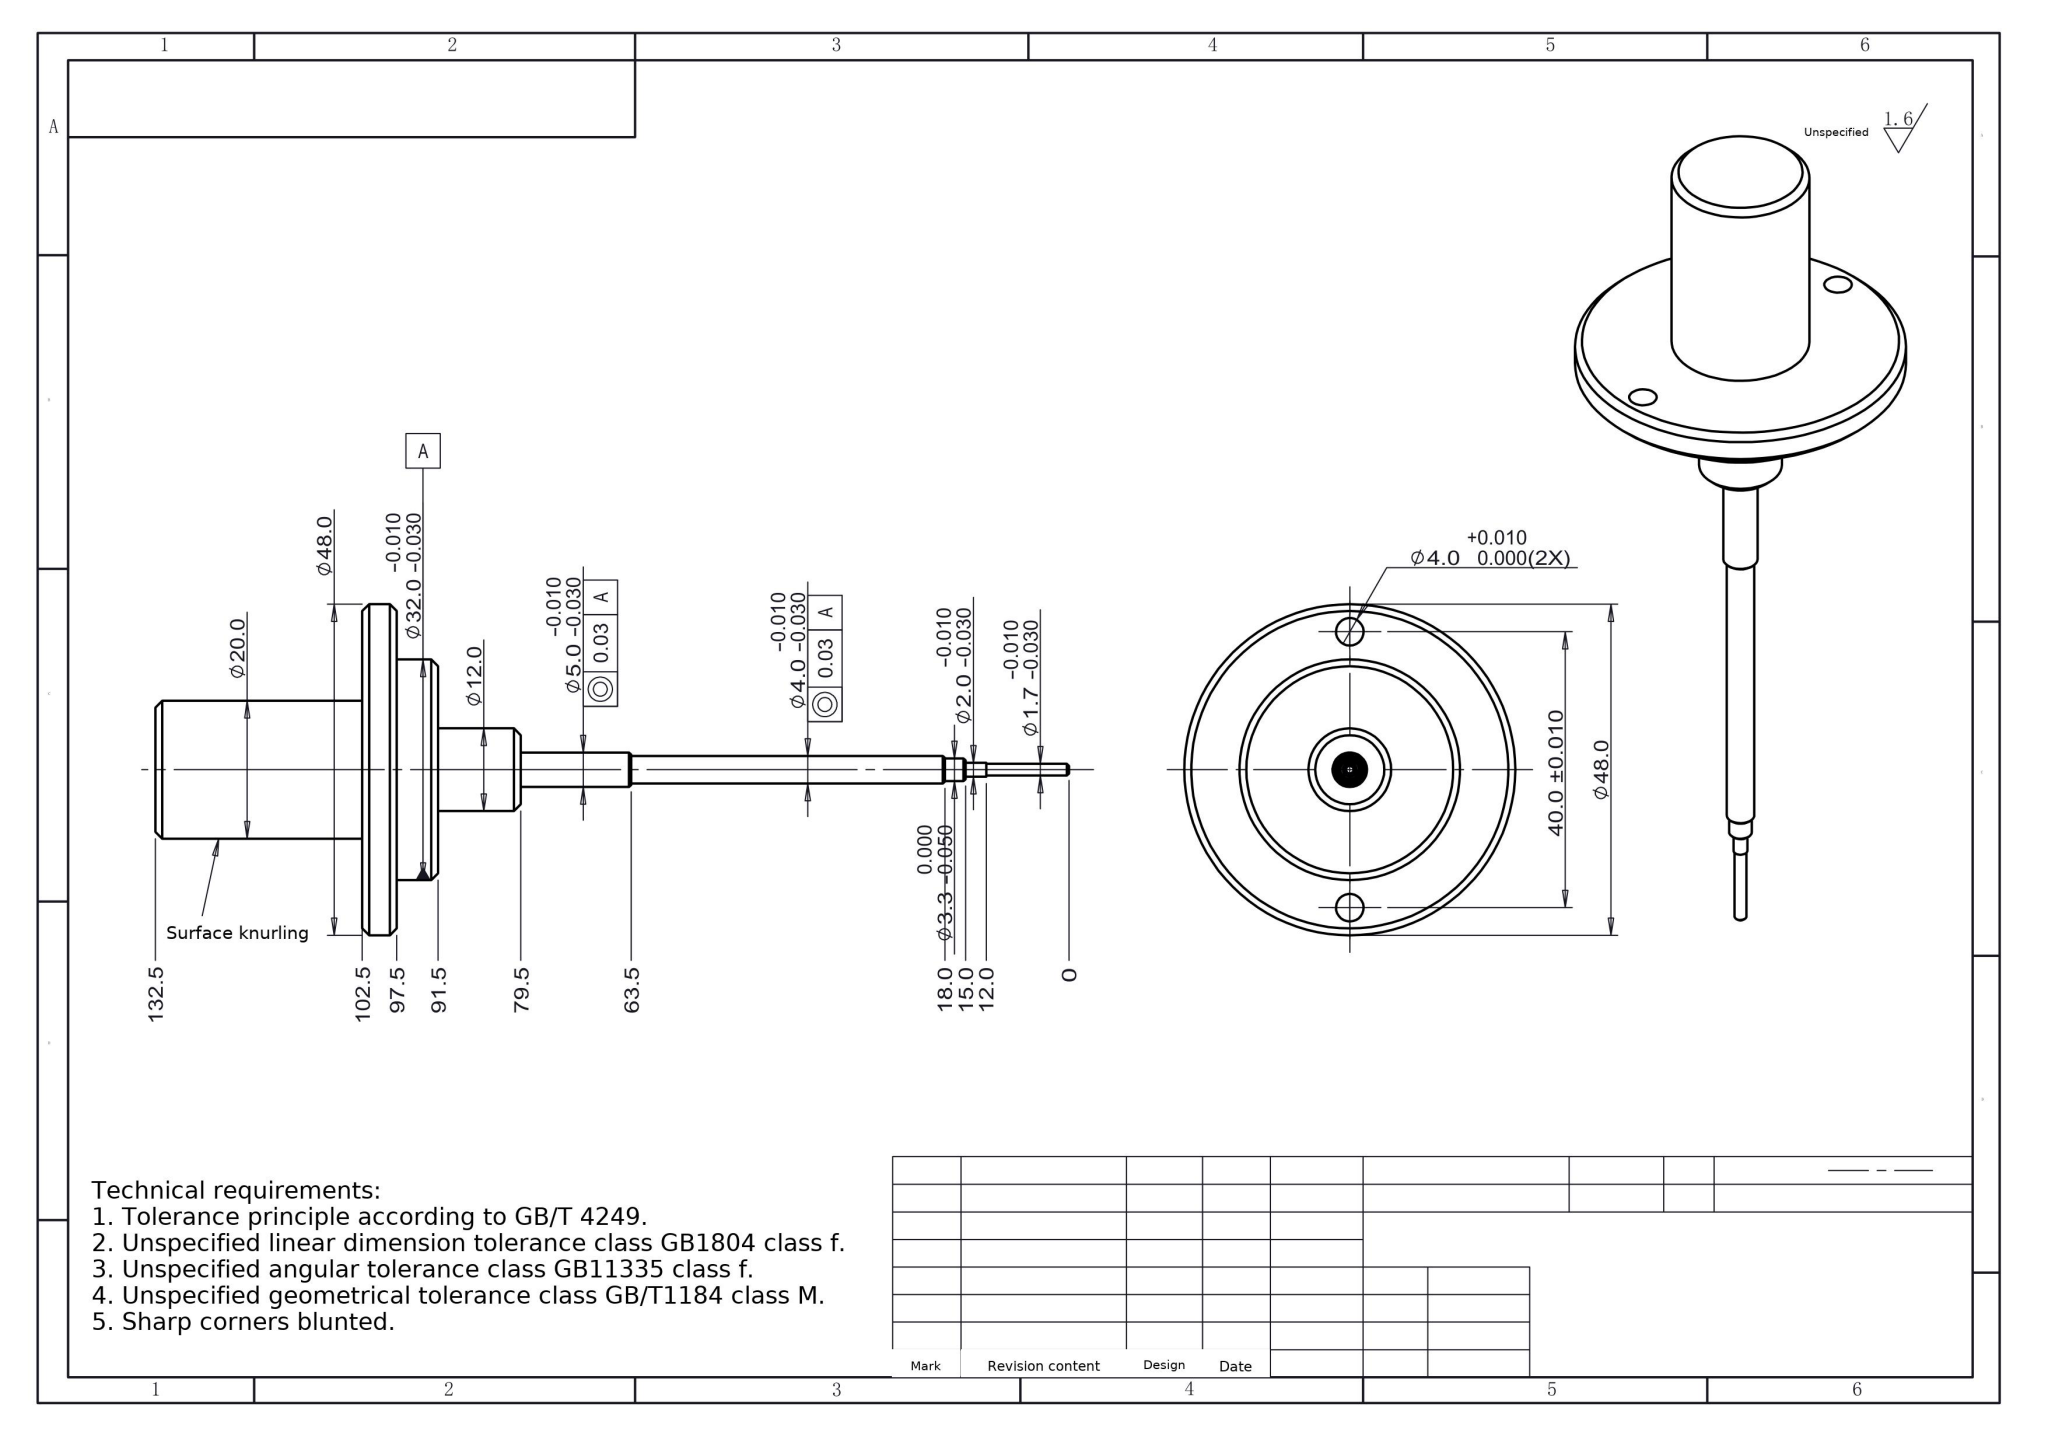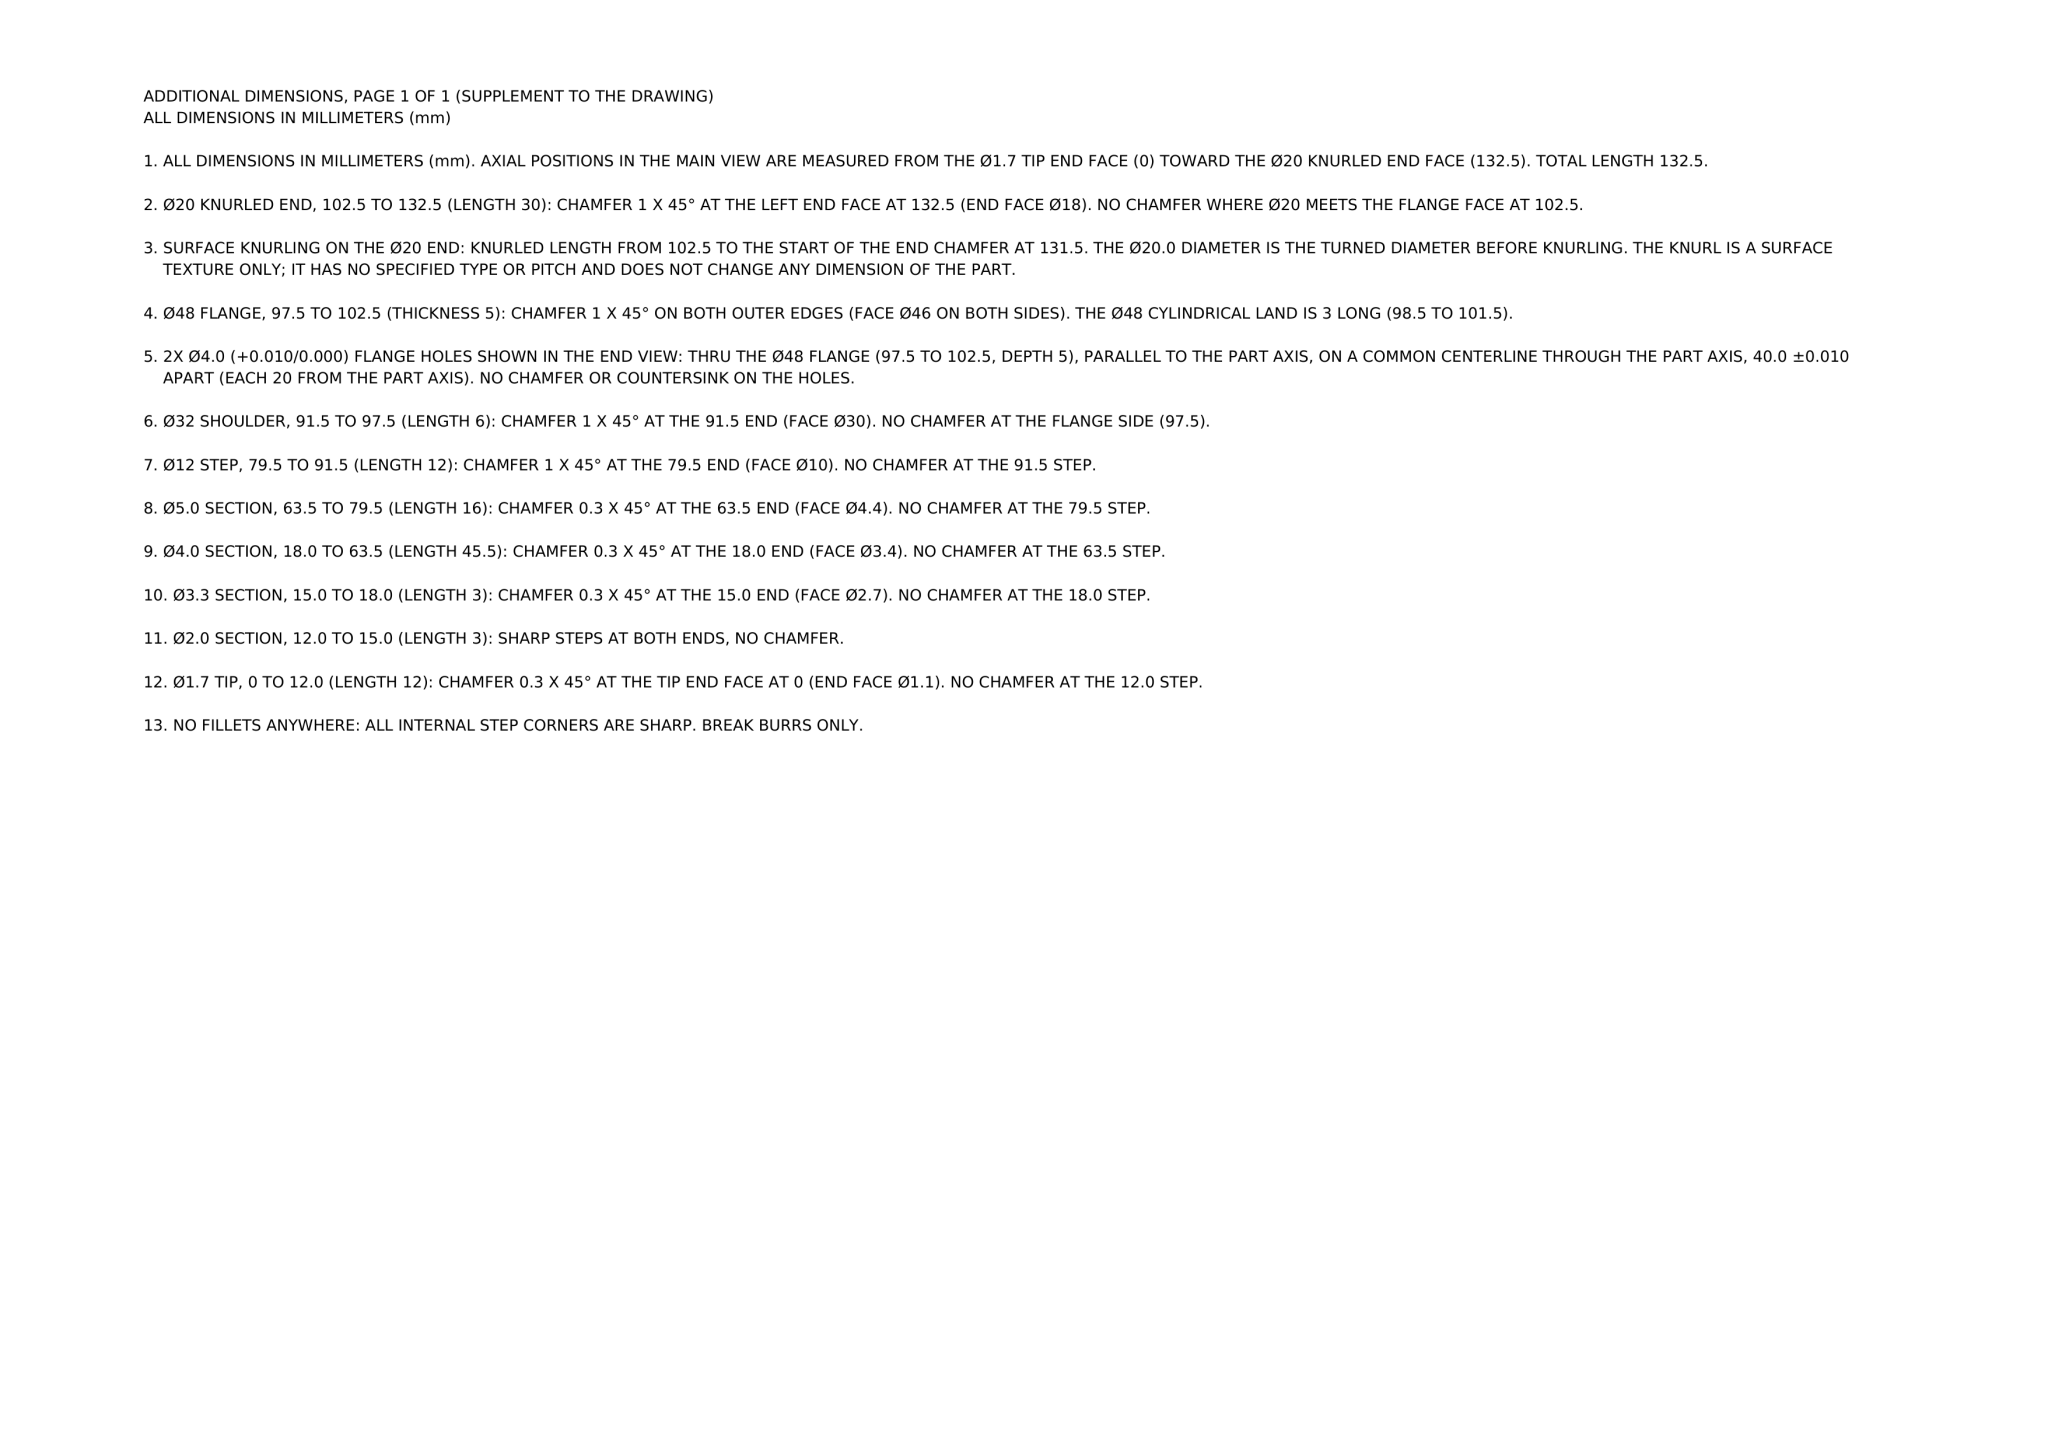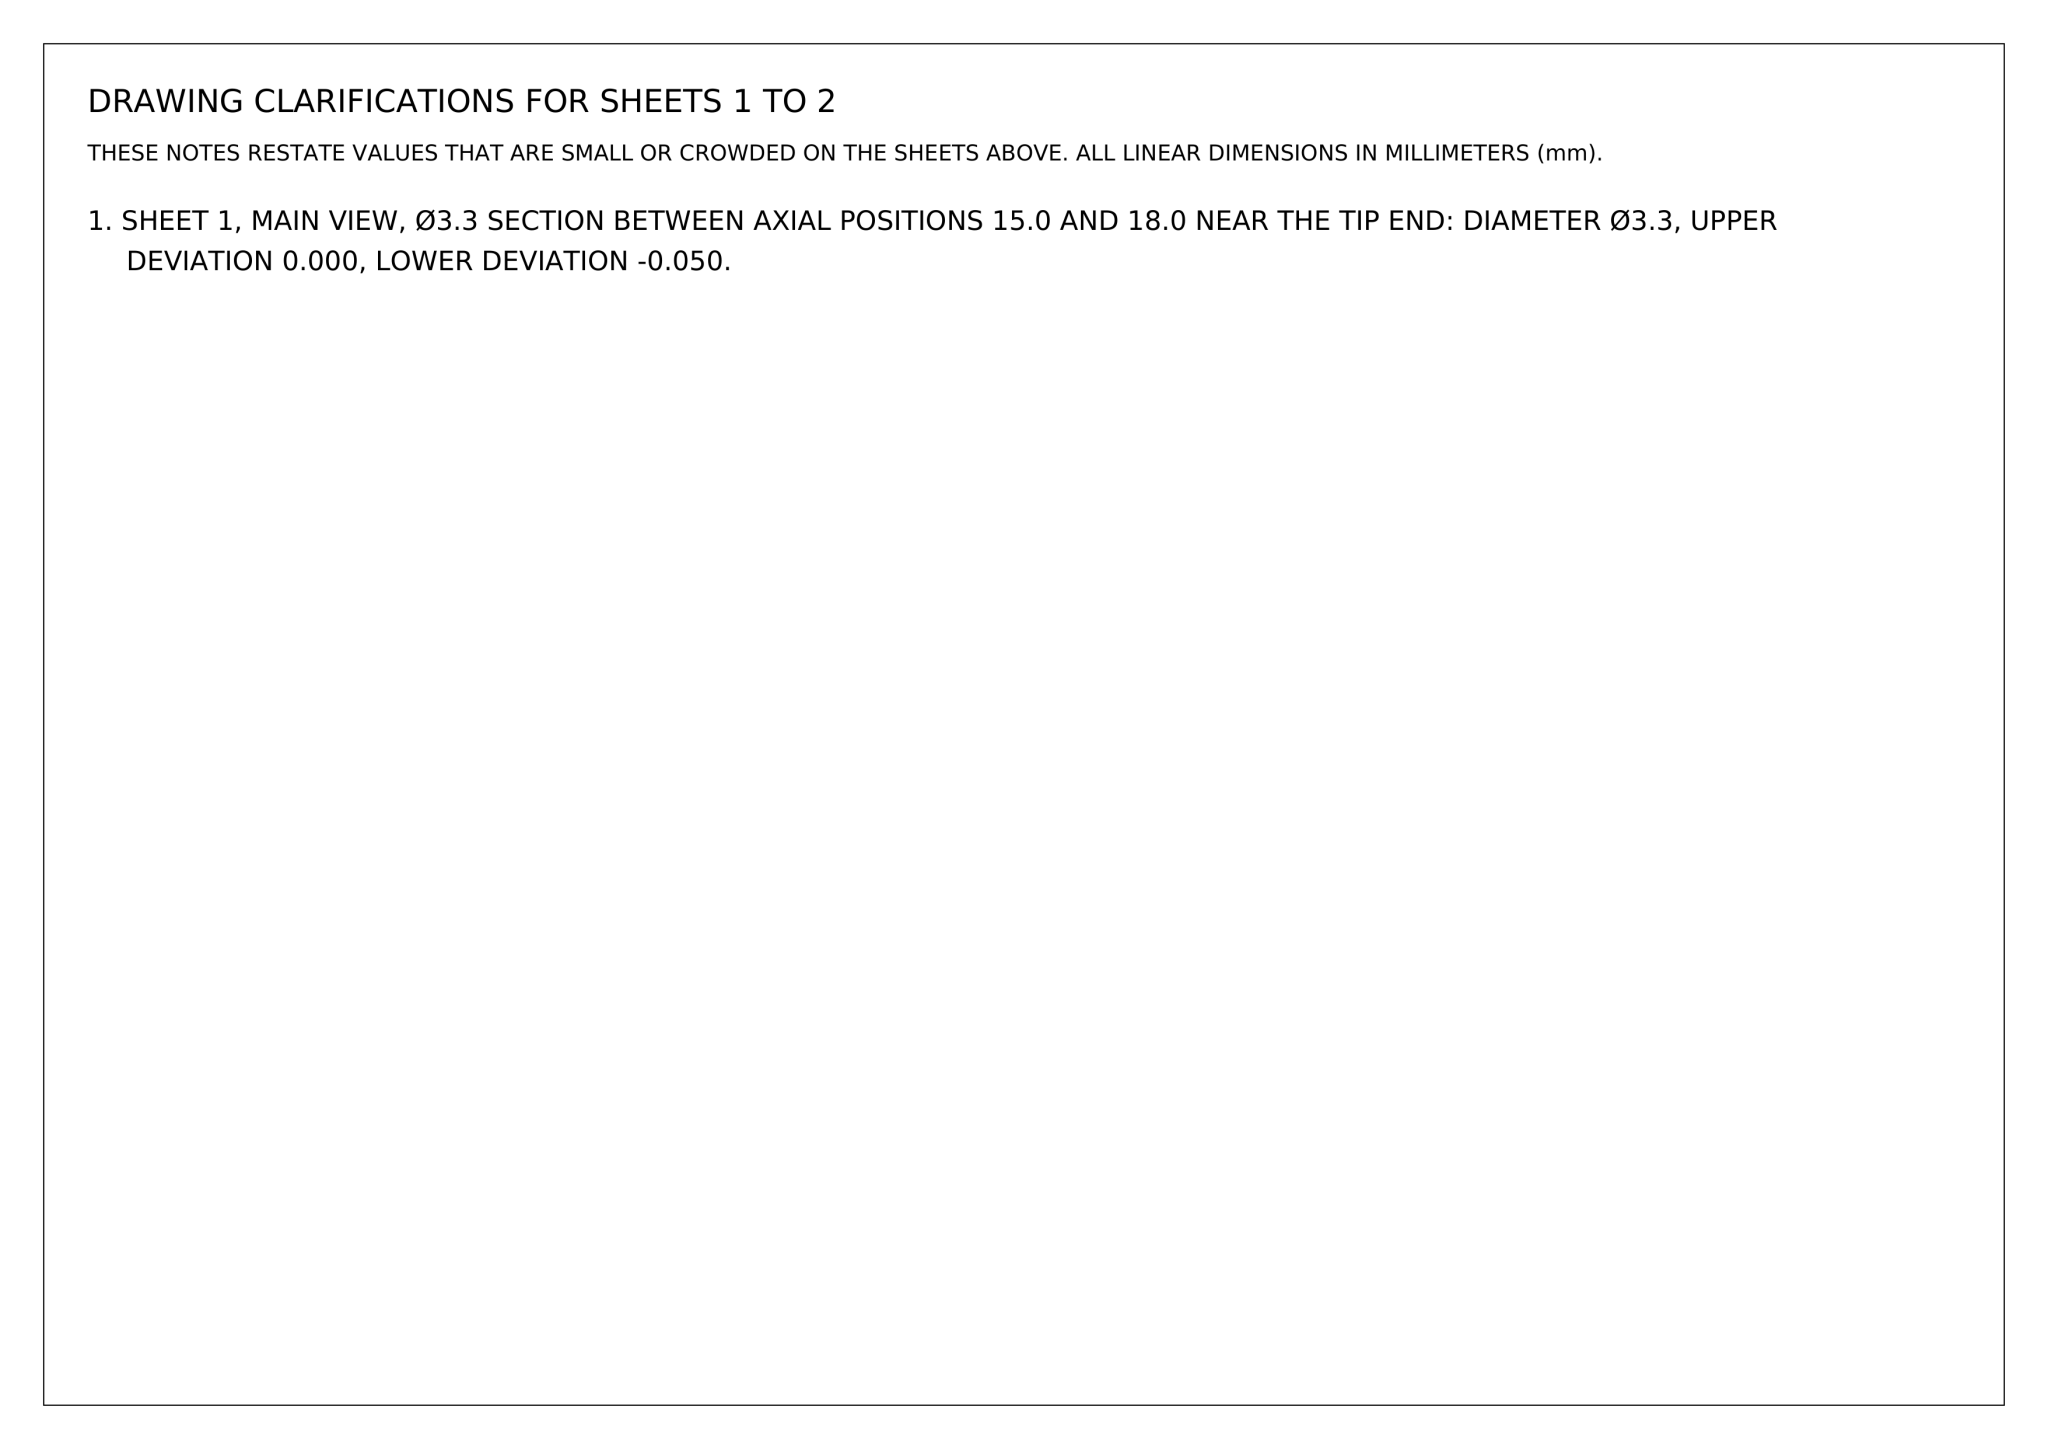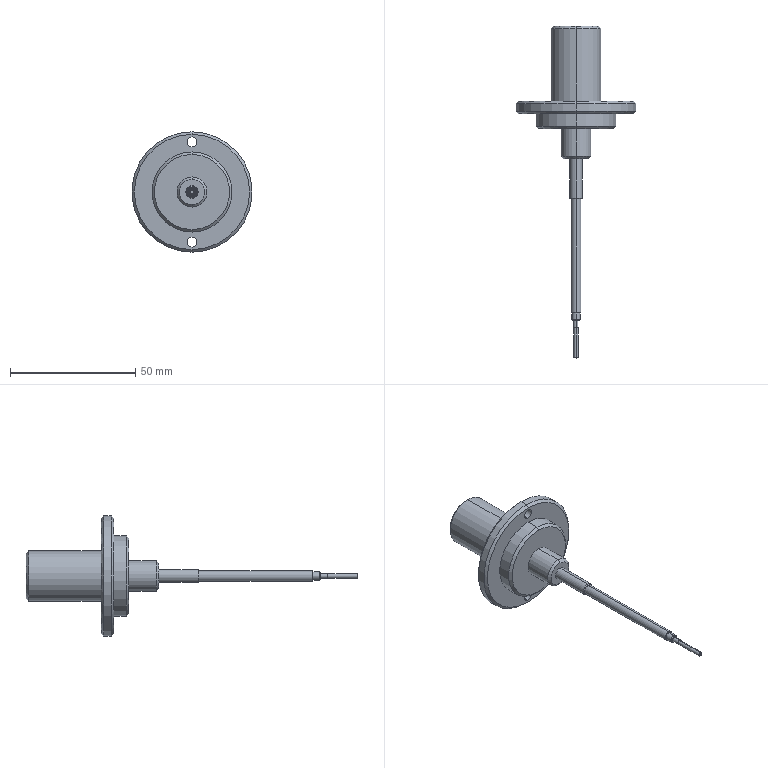Part | NX | mm | 1 solid | 50 faces | box 48 x 132.5 x 48 mm | volume 25230 mm3 | cylinder 22 | cone 18 | plane 10 | commonest cylinder face diameters 4 x6 2 x2 1.7 x2 3.3 x2 5 x2 12 x2 32 x2 48 x2